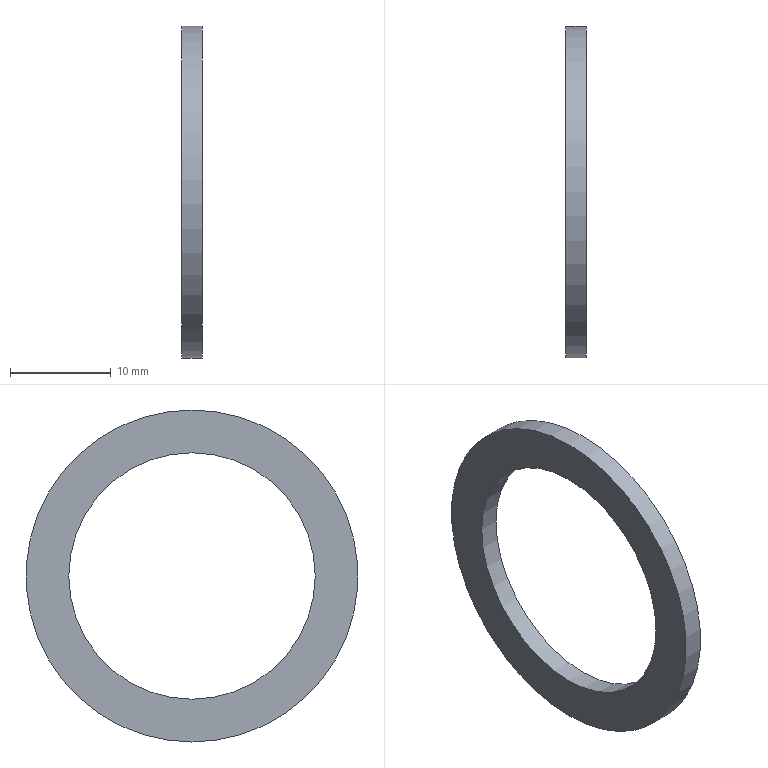Component | NX | WASHER | 1 solid | 4 faces | box 2 x 33 x 33 mm | volume 768 mm3 | cylinder 2 | plane 2 | commonest cylinder face diameters 33 x1 24.5 x1
STEP:
#1=CARTESIAN_POINT('',(0.,0.,0.));
#2=DIRECTION('',(0.,0.,1.));
#3=DIRECTION('',(1.,0.,0.));
#4=AXIS2_PLACEMENT_3D('',#1,#2,#3);
#5=CARTESIAN_POINT('',(88.295,-20.891,16.5));
#6=VERTEX_POINT('',#5);
#7=CARTESIAN_POINT('',(88.295,-20.891,0.));
#8=DIRECTION('',(1.,0.,0.));
#9=DIRECTION('',(0.,0.,1.));
#10=AXIS2_PLACEMENT_3D('',#7,#8,#9);
#11=CIRCLE('',#10,16.5);
#12=CARTESIAN_POINT('',(88.295,-20.891,0.));
#13=DIRECTION('',(-1.,0.,0.));
#14=DIRECTION('',(0.,0.,-1.));
#15=AXIS2_PLACEMENT_3D('',#12,#13,#14);
#16=CYLINDRICAL_SURFACE('',#15,16.5);
#17=CARTESIAN_POINT('',(9.425,0.));
#18=DIRECTION('',(-1.,0.));
#19=VECTOR('',#18,1.);
#20=LINE('',#17,#19);
#21=(GEOMETRIC_REPRESENTATION_CONTEXT(2)PARAMETRIC_REPRESENTATION_CONTEXT()REPRESENTATION_CONTEXT('',''));
#22=DEFINITIONAL_REPRESENTATION('',(#20),#21);
#23=PCURVE('',#16,#22);
#24=CARTESIAN_POINT('',(88.295,-20.891,0.));
#25=DIRECTION('',(1.,0.,0.));
#26=DIRECTION('',(0.,0.,1.));
#27=AXIS2_PLACEMENT_3D('',#24,#25,#26);
#28=PLANE('',#27);
#29=CARTESIAN_POINT('',(0.,0.));
#30=DIRECTION('',(1.,0.));
#31=AXIS2_PLACEMENT_2D('',#29,#30);
#32=CIRCLE('',#31,16.5);
#33=(GEOMETRIC_REPRESENTATION_CONTEXT(2)PARAMETRIC_REPRESENTATION_CONTEXT()REPRESENTATION_CONTEXT('',''));
#34=DEFINITIONAL_REPRESENTATION('',(#32),#33);
#35=PCURVE('',#28,#34);
#36=SURFACE_CURVE('',#11,(#23,#35),.PCURVE_S1.);
#37=EDGE_CURVE('',#6,#6,#36,.T.);
#38=ORIENTED_EDGE('',*,*,#37,.F.);
#39=CARTESIAN_POINT('',(86.295,-20.891,16.5));
#40=VERTEX_POINT('',#39);
#41=CARTESIAN_POINT('',(88.295,-20.891,16.5));
#42=CARTESIAN_POINT('',(86.295,-20.891,16.5));
#43=B_SPLINE_CURVE_WITH_KNOTS('',1,(#41,#42),.UNSPECIFIED.,.F.,.F.,(2,2),(0.,2.),.PIECEWISE_BEZIER_KNOTS.);
#44=CARTESIAN_POINT('',(9.425,0.));
#45=DIRECTION('',(0.,1.));
#46=VECTOR('',#45,1.);
#47=LINE('',#44,#46);
#48=(GEOMETRIC_REPRESENTATION_CONTEXT(2)PARAMETRIC_REPRESENTATION_CONTEXT()REPRESENTATION_CONTEXT('',''));
#49=DEFINITIONAL_REPRESENTATION('',(#47),#48);
#50=PCURVE('',#16,#49);
#51=CARTESIAN_POINT('',(3.142,0.));
#52=DIRECTION('',(0.,1.));
#53=VECTOR('',#52,1.);
#54=LINE('',#51,#53);
#55=(GEOMETRIC_REPRESENTATION_CONTEXT(2)PARAMETRIC_REPRESENTATION_CONTEXT()REPRESENTATION_CONTEXT('',''));
#56=DEFINITIONAL_REPRESENTATION('',(#54),#55);
#57=PCURVE('',#16,#56);
#58=SEAM_CURVE('',#43,(#50,#57),.PCURVE_S1.);
#59=EDGE_CURVE('',#6,#40,#58,.T.);
#60=ORIENTED_EDGE('',*,*,#59,.T.);
#61=CARTESIAN_POINT('',(86.295,-20.891,0.));
#62=DIRECTION('',(1.,0.,0.));
#63=DIRECTION('',(0.,0.,1.));
#64=AXIS2_PLACEMENT_3D('',#61,#62,#63);
#65=CIRCLE('',#64,16.5);
#66=CARTESIAN_POINT('',(9.425,2.));
#67=DIRECTION('',(-1.,0.));
#68=VECTOR('',#67,1.);
#69=LINE('',#66,#68);
#70=(GEOMETRIC_REPRESENTATION_CONTEXT(2)PARAMETRIC_REPRESENTATION_CONTEXT()REPRESENTATION_CONTEXT('',''));
#71=DEFINITIONAL_REPRESENTATION('',(#69),#70);
#72=PCURVE('',#16,#71);
#73=CARTESIAN_POINT('',(86.295,-20.891,0.));
#74=DIRECTION('',(1.,0.,0.));
#75=DIRECTION('',(0.,0.,1.));
#76=AXIS2_PLACEMENT_3D('',#73,#74,#75);
#77=PLANE('',#76);
#78=CARTESIAN_POINT('',(0.,0.));
#79=DIRECTION('',(1.,0.));
#80=AXIS2_PLACEMENT_2D('',#78,#79);
#81=CIRCLE('',#80,16.5);
#82=(GEOMETRIC_REPRESENTATION_CONTEXT(2)PARAMETRIC_REPRESENTATION_CONTEXT()REPRESENTATION_CONTEXT('',''));
#83=DEFINITIONAL_REPRESENTATION('',(#81),#82);
#84=PCURVE('',#77,#83);
#85=SURFACE_CURVE('',#65,(#72,#84),.PCURVE_S1.);
#86=EDGE_CURVE('',#40,#40,#85,.T.);
#87=ORIENTED_EDGE('',*,*,#86,.T.);
#88=ORIENTED_EDGE('',*,*,#59,.F.);
#89=EDGE_LOOP('',(#38,#60,#87,#88));
#90=FACE_BOUND('',#89,.T.);
#91=ADVANCED_FACE('',(#90),#16,.T.);
#92=CARTESIAN_POINT('',(88.295,-20.891,12.25));
#93=VERTEX_POINT('',#92);
#94=CARTESIAN_POINT('',(88.295,-20.891,0.));
#95=DIRECTION('',(1.,0.,0.));
#96=DIRECTION('',(0.,0.,1.));
#97=AXIS2_PLACEMENT_3D('',#94,#95,#96);
#98=CIRCLE('',#97,12.25);
#99=CARTESIAN_POINT('',(88.295,-20.891,0.));
#100=DIRECTION('',(-1.,0.,0.));
#101=DIRECTION('',(0.,0.,-1.));
#102=AXIS2_PLACEMENT_3D('',#99,#100,#101);
#103=CYLINDRICAL_SURFACE('',#102,12.25);
#104=CARTESIAN_POINT('',(9.425,0.));
#105=DIRECTION('',(-1.,0.));
#106=VECTOR('',#105,1.);
#107=LINE('',#104,#106);
#108=(GEOMETRIC_REPRESENTATION_CONTEXT(2)PARAMETRIC_REPRESENTATION_CONTEXT()REPRESENTATION_CONTEXT('',''));
#109=DEFINITIONAL_REPRESENTATION('',(#107),#108);
#110=PCURVE('',#103,#109);
#111=CARTESIAN_POINT('',(0.,0.));
#112=DIRECTION('',(1.,0.));
#113=AXIS2_PLACEMENT_2D('',#111,#112);
#114=CIRCLE('',#113,12.25);
#115=(GEOMETRIC_REPRESENTATION_CONTEXT(2)PARAMETRIC_REPRESENTATION_CONTEXT()REPRESENTATION_CONTEXT('',''));
#116=DEFINITIONAL_REPRESENTATION('',(#114),#115);
#117=PCURVE('',#28,#116);
#118=SURFACE_CURVE('',#98,(#110,#117),.PCURVE_S1.);
#119=EDGE_CURVE('',#93,#93,#118,.T.);
#120=ORIENTED_EDGE('',*,*,#119,.F.);
#121=CARTESIAN_POINT('',(86.295,-20.891,12.25));
#122=VERTEX_POINT('',#121);
#123=CARTESIAN_POINT('',(88.295,-20.891,12.25));
#124=CARTESIAN_POINT('',(86.295,-20.891,12.25));
#125=B_SPLINE_CURVE_WITH_KNOTS('',1,(#123,#124),.UNSPECIFIED.,.F.,.F.,(2,2),(0.,2.),.PIECEWISE_BEZIER_KNOTS.);
#126=CARTESIAN_POINT('',(9.425,0.));
#127=DIRECTION('',(0.,1.));
#128=VECTOR('',#127,1.);
#129=LINE('',#126,#128);
#130=(GEOMETRIC_REPRESENTATION_CONTEXT(2)PARAMETRIC_REPRESENTATION_CONTEXT()REPRESENTATION_CONTEXT('',''));
#131=DEFINITIONAL_REPRESENTATION('',(#129),#130);
#132=PCURVE('',#103,#131);
#133=CARTESIAN_POINT('',(3.142,0.));
#134=DIRECTION('',(0.,1.));
#135=VECTOR('',#134,1.);
#136=LINE('',#133,#135);
#137=(GEOMETRIC_REPRESENTATION_CONTEXT(2)PARAMETRIC_REPRESENTATION_CONTEXT()REPRESENTATION_CONTEXT('',''));
#138=DEFINITIONAL_REPRESENTATION('',(#136),#137);
#139=PCURVE('',#103,#138);
#140=SEAM_CURVE('',#125,(#132,#139),.PCURVE_S1.);
#141=EDGE_CURVE('',#93,#122,#140,.T.);
#142=ORIENTED_EDGE('',*,*,#141,.T.);
#143=CARTESIAN_POINT('',(86.295,-20.891,0.));
#144=DIRECTION('',(1.,0.,0.));
#145=DIRECTION('',(0.,0.,1.));
#146=AXIS2_PLACEMENT_3D('',#143,#144,#145);
#147=CIRCLE('',#146,12.25);
#148=CARTESIAN_POINT('',(9.425,2.));
#149=DIRECTION('',(-1.,0.));
#150=VECTOR('',#149,1.);
#151=LINE('',#148,#150);
#152=(GEOMETRIC_REPRESENTATION_CONTEXT(2)PARAMETRIC_REPRESENTATION_CONTEXT()REPRESENTATION_CONTEXT('',''));
#153=DEFINITIONAL_REPRESENTATION('',(#151),#152);
#154=PCURVE('',#103,#153);
#155=CARTESIAN_POINT('',(0.,0.));
#156=DIRECTION('',(1.,0.));
#157=AXIS2_PLACEMENT_2D('',#155,#156);
#158=CIRCLE('',#157,12.25);
#159=(GEOMETRIC_REPRESENTATION_CONTEXT(2)PARAMETRIC_REPRESENTATION_CONTEXT()REPRESENTATION_CONTEXT('',''));
#160=DEFINITIONAL_REPRESENTATION('',(#158),#159);
#161=PCURVE('',#77,#160);
#162=SURFACE_CURVE('',#147,(#154,#161),.PCURVE_S1.);
#163=EDGE_CURVE('',#122,#122,#162,.T.);
#164=ORIENTED_EDGE('',*,*,#163,.T.);
#165=ORIENTED_EDGE('',*,*,#141,.F.);
#166=EDGE_LOOP('',(#120,#142,#164,#165));
#167=FACE_BOUND('',#166,.F.);
#168=ADVANCED_FACE('',(#167),#103,.F.);
#169=ORIENTED_EDGE('',*,*,#37,.T.);
#170=EDGE_LOOP('',(#169));
#171=FACE_BOUND('',#170,.T.);
#172=ORIENTED_EDGE('',*,*,#119,.F.);
#173=EDGE_LOOP('',(#172));
#174=FACE_BOUND('',#173,.T.);
#175=ADVANCED_FACE('',(#171,#174),#28,.T.);
#176=ORIENTED_EDGE('',*,*,#86,.F.);
#177=EDGE_LOOP('',(#176));
#178=FACE_BOUND('',#177,.T.);
#179=ORIENTED_EDGE('',*,*,#163,.T.);
#180=EDGE_LOOP('',(#179));
#181=FACE_BOUND('',#180,.T.);
#182=ADVANCED_FACE('',(#178,#181),#77,.F.);
#183=CLOSED_SHELL('',(#91,#168,#175,#182));
#184=MANIFOLD_SOLID_BREP('',#183);
#185=(LENGTH_UNIT()NAMED_UNIT(*)SI_UNIT(.MILLI.,.METRE.));
#186=UNCERTAINTY_MEASURE_WITH_UNIT(LENGTH_MEASURE(0.00001),#185,'','');
#187=(NAMED_UNIT(*)PLANE_ANGLE_UNIT()SI_UNIT($,.RADIAN.));
#188=(NAMED_UNIT(*)SI_UNIT($,.STERADIAN.)SOLID_ANGLE_UNIT());
#189=(GEOMETRIC_REPRESENTATION_CONTEXT(3)GLOBAL_UNCERTAINTY_ASSIGNED_CONTEXT((#186))GLOBAL_UNIT_ASSIGNED_CONTEXT((#185,#187,#188))REPRESENTATION_CONTEXT('',''));
#190=ADVANCED_BREP_SHAPE_REPRESENTATION('',(#4,#184),#189);